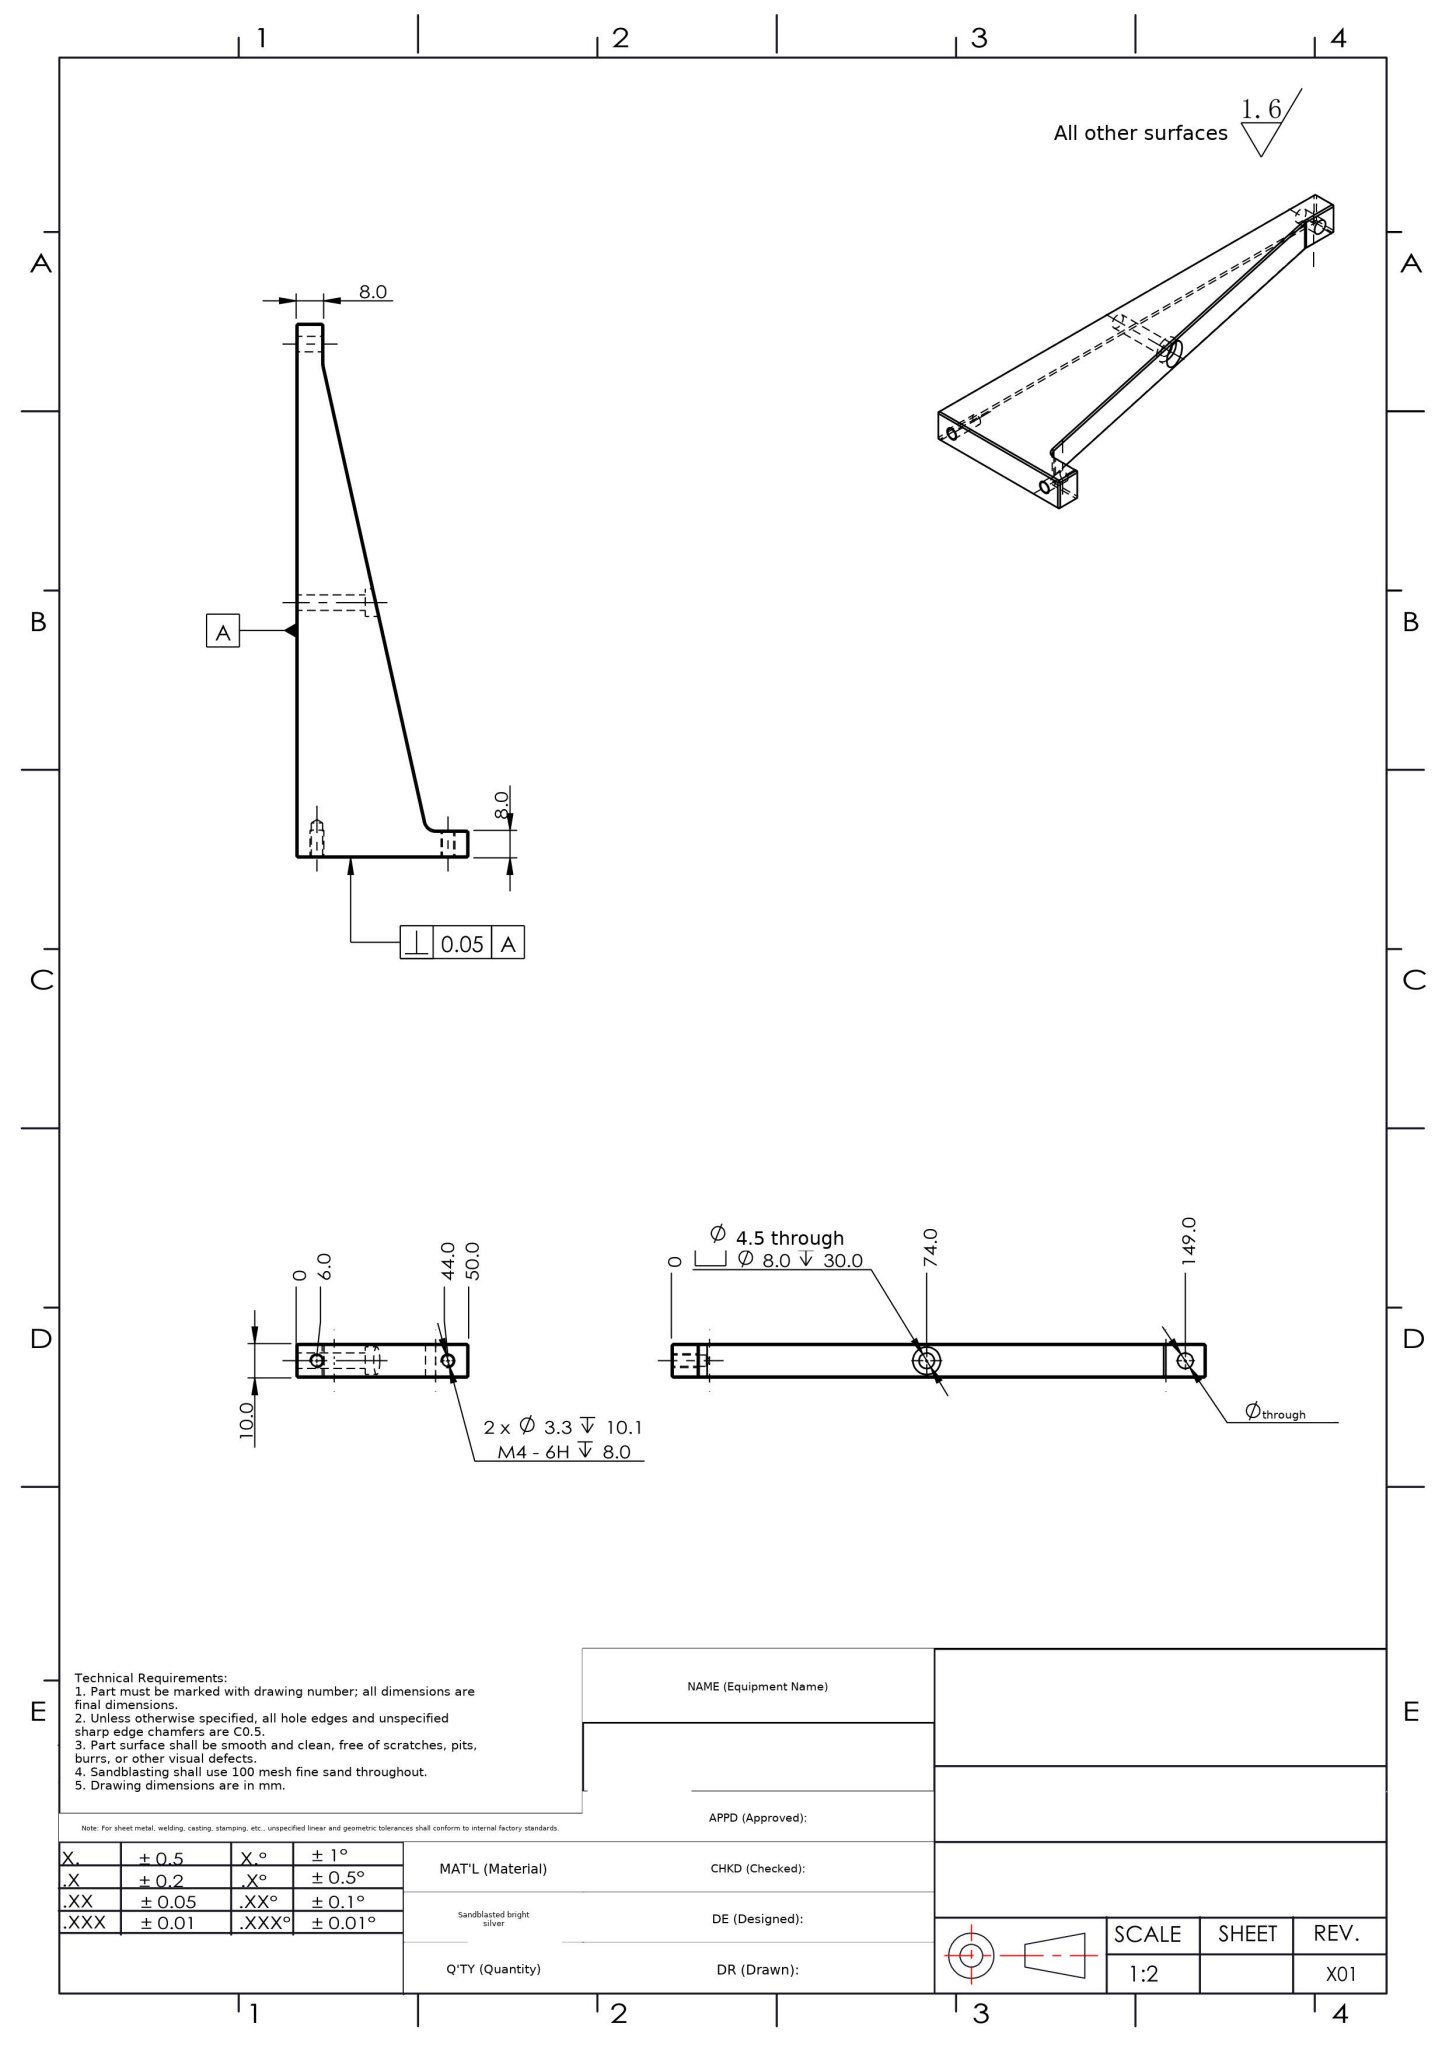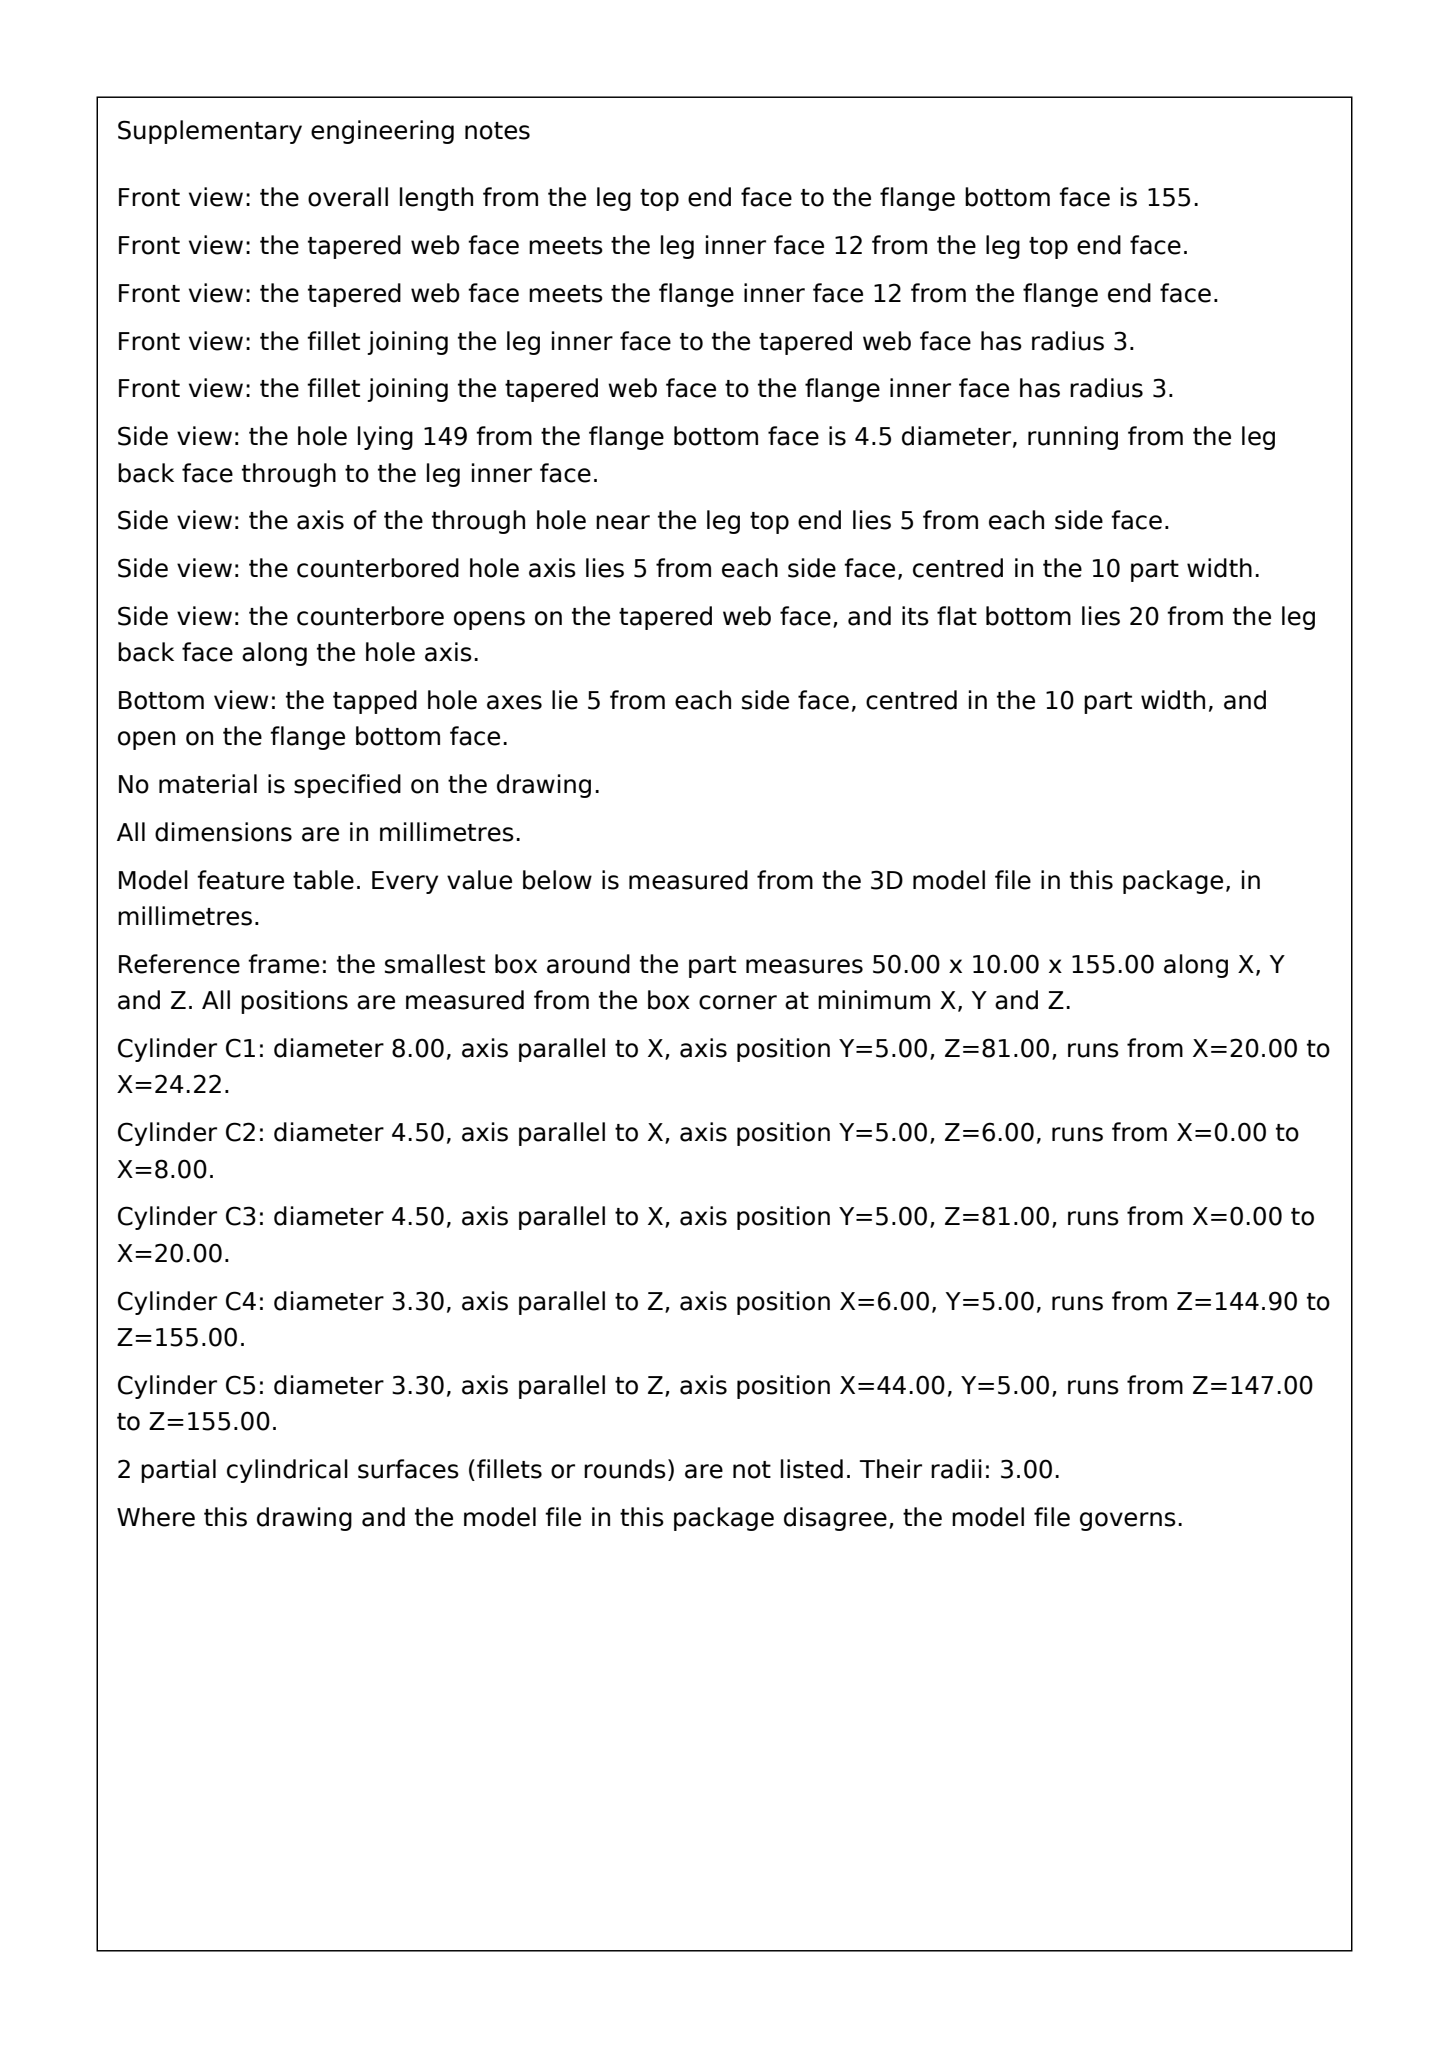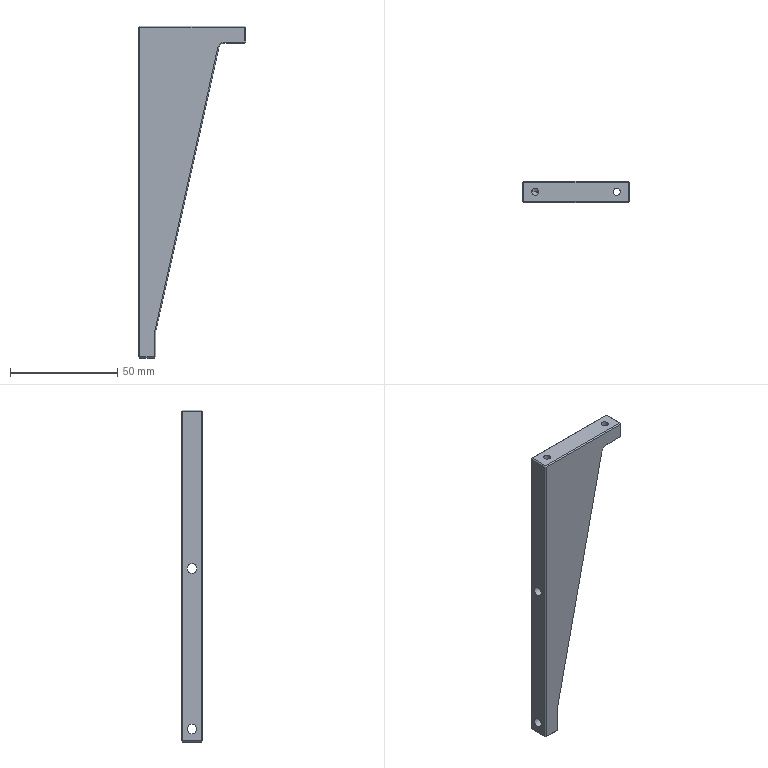Part | SolidWorks | mm | 1 solid | 57 faces | box 50 x 10 x 155 mm | volume 35150 mm3 | plane 39 | cylinder 12 | cone 6 | commonest cylinder face diameters 4.5 x4 3.3 x4 8 x2 6 x2
Drawing notes:
2X Ø6.0 DP 9.0 IN 50X155 FACE: X11.0/Z143.33 & X40.41/Z11.0 | from the solid: cyl Ø6.0 axis y, pos (11.0,11.67) & (40.41,144.0), L=9.0; Z given from drawing 0 datum (155-11.67=143.33, 155-144=11.0)
HOLE AT 149.0: Ø4.5 THRU (8.0 WALL) | from the solid: cyl Ø4.5 axis x at z=6.0 (=149.0 from drawing 0 datum), length 8.0
4X Ø7.0 X 90° CSK ON Ø4.5 CROSS HOLES, EA END | from the solid: cones[90.0, ref_dia 7.0] count 4 on the Ø4.5 x-axis holes
AT 74.0: Ø4.5 THRU 20.0, CBORE Ø8.0 DP 4.22 FROM EA FACE | from the solid: cyl Ø4.5 axis x at z=81.0 L=20.0; 2X cyl Ø8.0 same axis L=4.22 (one per face)
build123d program:
from build123d import *

# Parameters (mm, degrees)
BOSS_EXTRUDE1_DEPTH                             = 10
FILLET1_R                                       = 3
M4_TAPPED_HOLE1_D                               = 3.3
M4_TAPPED_HOLE1_DEPTH                           = 10.1
M4_TAPPED_HOLE1_TIP                             = 0.9914
M4_HEX_SOCKET_HEAD_CAP_SCREW_CBORE1_D           = 4.5
M4_HEX_SOCKET_HEAD_CAP_SCREW_CBORE1_CBORE_D     = 8
M4_HEX_SOCKET_HEAD_CAP_SCREW_CBORE1_CBORE_DEPTH = 30
CHAMFER1_SIZE                                   = 0.5


with BuildPart() as part:
    # Sketch1 → Boss-Extrude1 (new body)
    with BuildSketch(Plane(origin=(0, 0, 0), x_dir=(1, 0, 0), z_dir=(0, 1, 0))):
        Polygon((0, 0), (8, 0), (8, -12), (38, -147), (50, -147), (50, -155), (0, -155), align=None)
    extrude(amount=BOSS_EXTRUDE1_DEPTH)

    # Fillet1
    fillet1_edges = [part.edges().sort_by_distance(p)[0] for p in [
        (8, 5, 12),
        (38, 5, 147),
    ]]
    fillet(fillet1_edges, radius=FILLET1_R)

    # M4 Tapped Hole1
    with Locations(Plane.XY.offset(155)):
        with Locations((44, 5), (6, 5)):
            Hole(M4_TAPPED_HOLE1_D / 2, depth=M4_TAPPED_HOLE1_DEPTH)
            with Locations((0, 0, -(M4_TAPPED_HOLE1_DEPTH + M4_TAPPED_HOLE1_TIP / 2))):  # 118° drill point
                Cone(0, M4_TAPPED_HOLE1_D / 2, M4_TAPPED_HOLE1_TIP, mode=Mode.SUBTRACT)

    # M4 Hex Socket Head Cap Screw CBORE1 (through all)
    with Locations(Plane(origin=(50, 0, 0), x_dir=(0, 0, -1), z_dir=(1, 0, 0))):
        with Locations((-81, 5), (-6, 5)):
            CounterBoreHole(M4_HEX_SOCKET_HEAD_CAP_SCREW_CBORE1_D / 2, M4_HEX_SOCKET_HEAD_CAP_SCREW_CBORE1_CBORE_D / 2, M4_HEX_SOCKET_HEAD_CAP_SCREW_CBORE1_CBORE_DEPTH)

    # Chamfer1
    chamfer1_edges = [part.edges().sort_by_distance(p)[0] for p in [
        (50, 10, 151),
        (0, 5, 0),
        (8, 5, 0),
        (50, 5, 147),
        (50, 5, 155),
        (0, 5, 155),
        (45.203, 10, 147),
        (8, 0, 5.835),
        (8, 10, 5.835),
        (4, 10, 0),
        (22.775, 0, 78.486),
        (22.775, 10, 78.486),
        (8.018, 0, 11.998),
        (8.018, 10, 11.998),
        (38.529, 0, 146.34),
        (38.529, 10, 146.34),
        (0, 10, 77.5),
        (4, 0, 0),
        (25, 10, 155),
        (45.203, 0, 147),
        (50, 0, 151),
        (25, 0, 155),
        (0, 0, 77.5),
    ]]
    chamfer(chamfer1_edges, length=CHAMFER1_SIZE)


solid = part.part